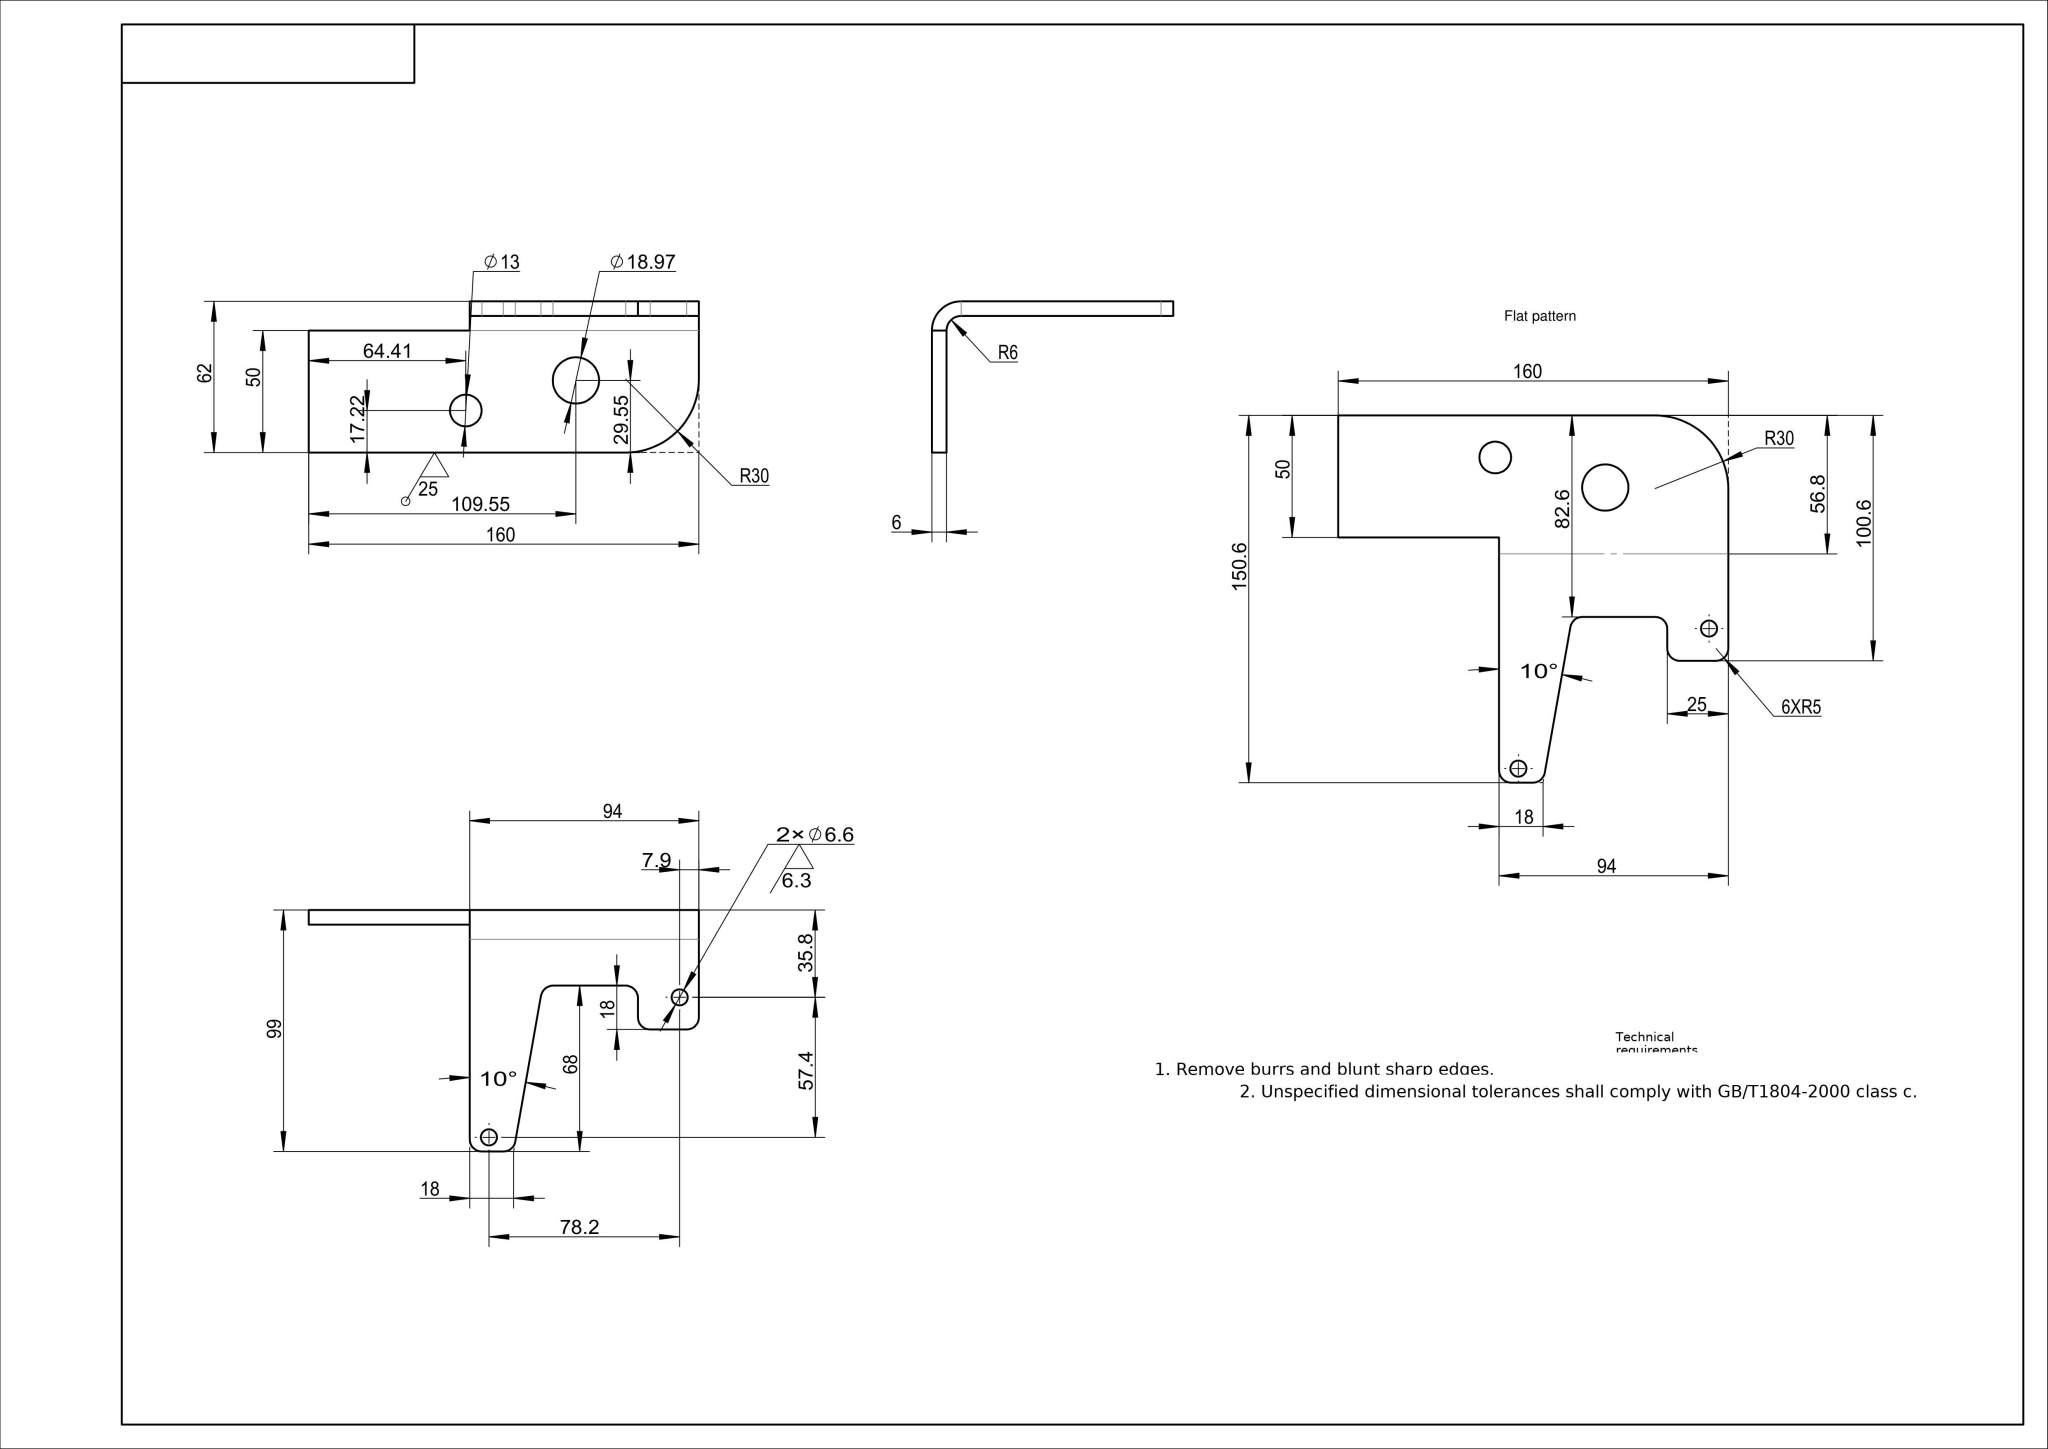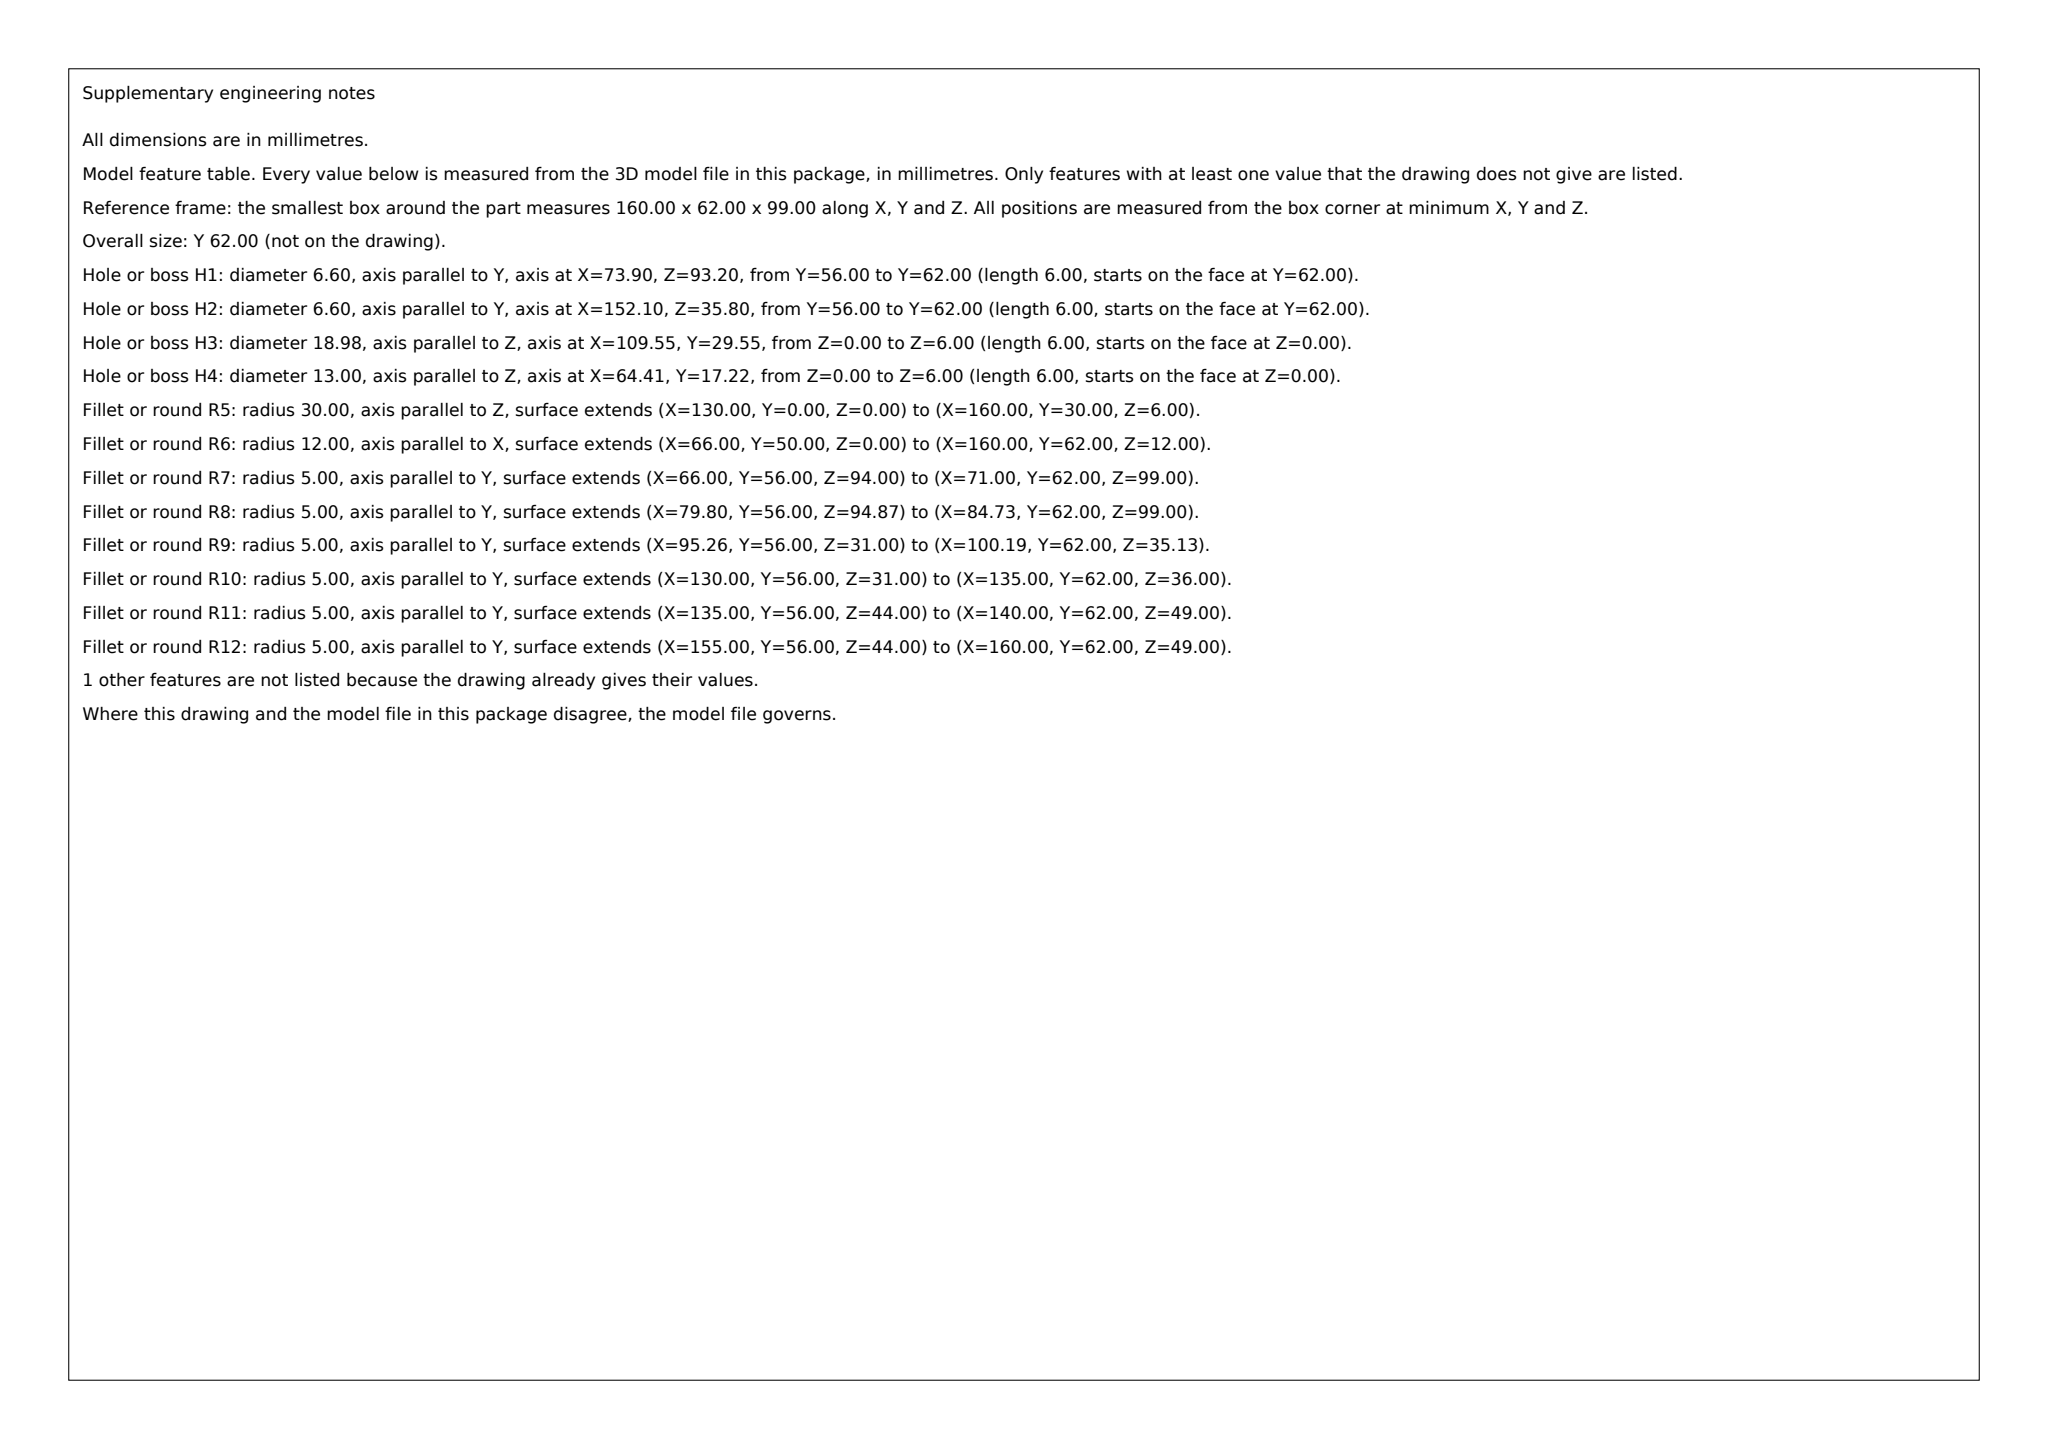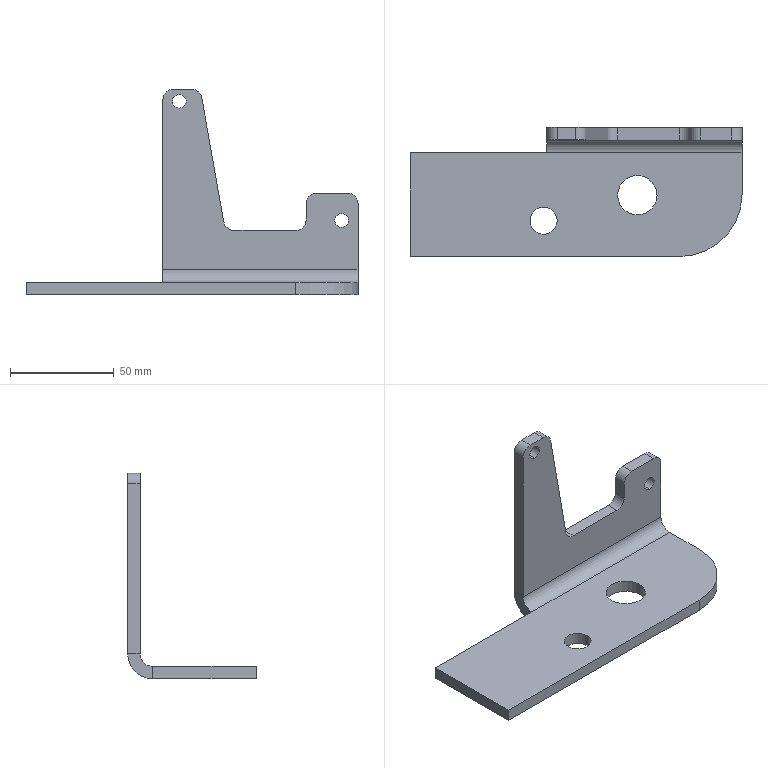Part | SolidWorks | mm | 1 solid | 34 faces | box 160 x 62 x 99 mm | volume 75053 mm3 | cylinder 17 | plane 17 | commonest cylinder face diameters 10 x6 6.6 x4 12.999 x2 18.975 x2 24 x1 12 x1 60 x1